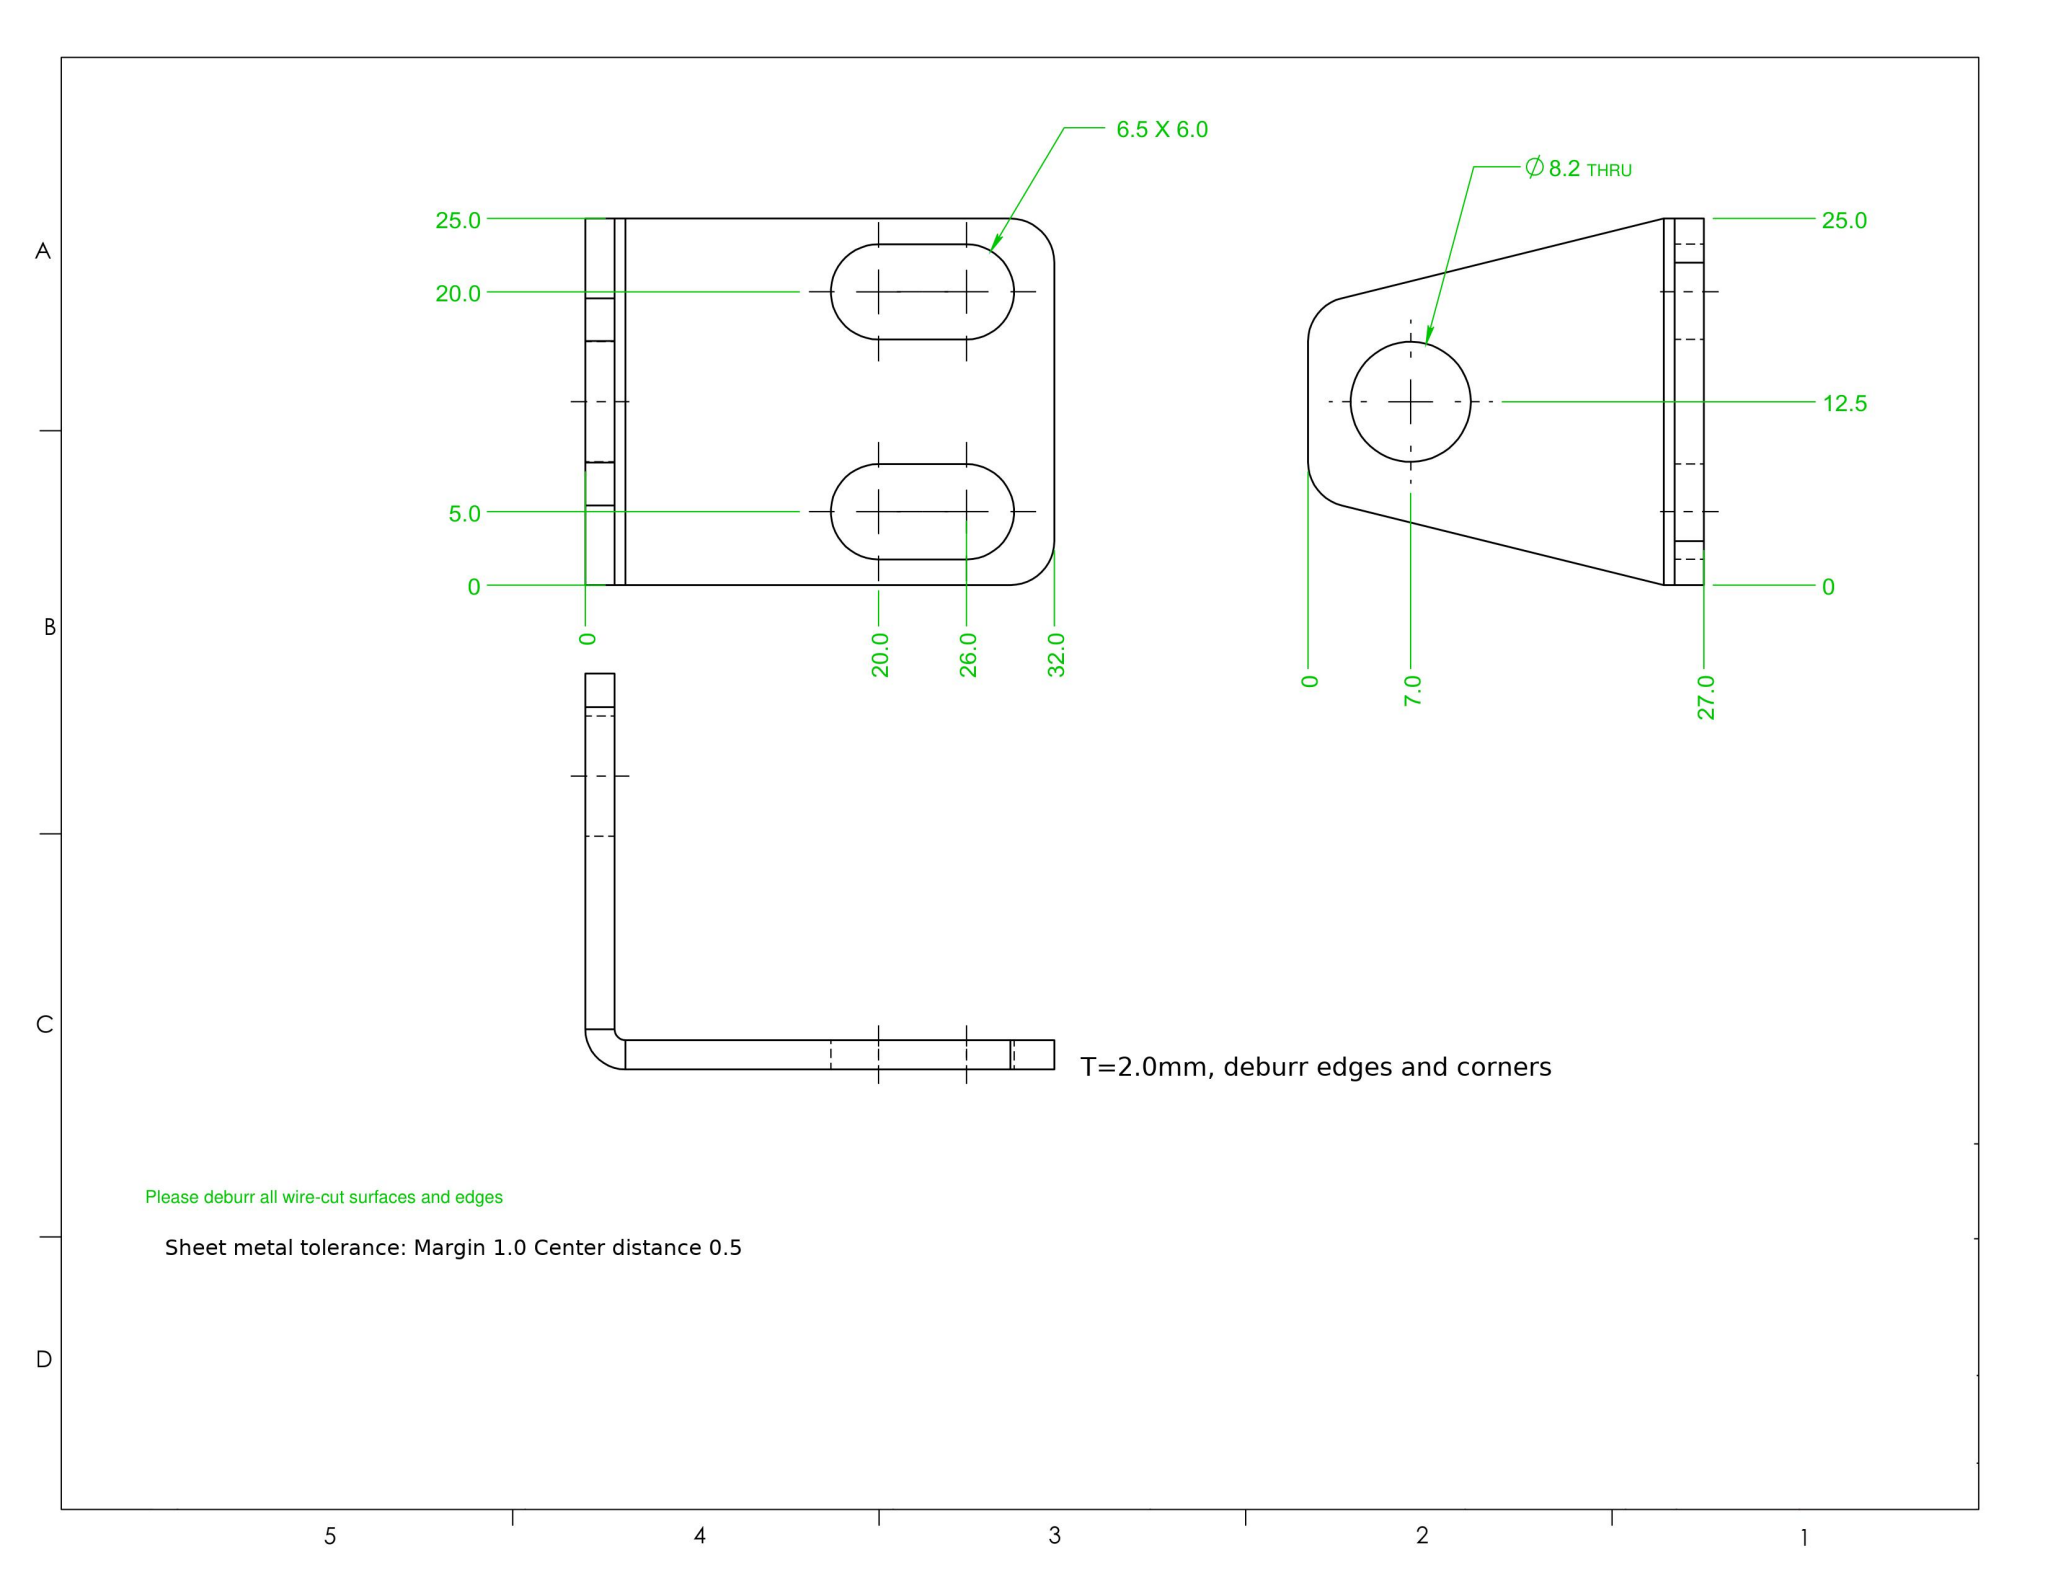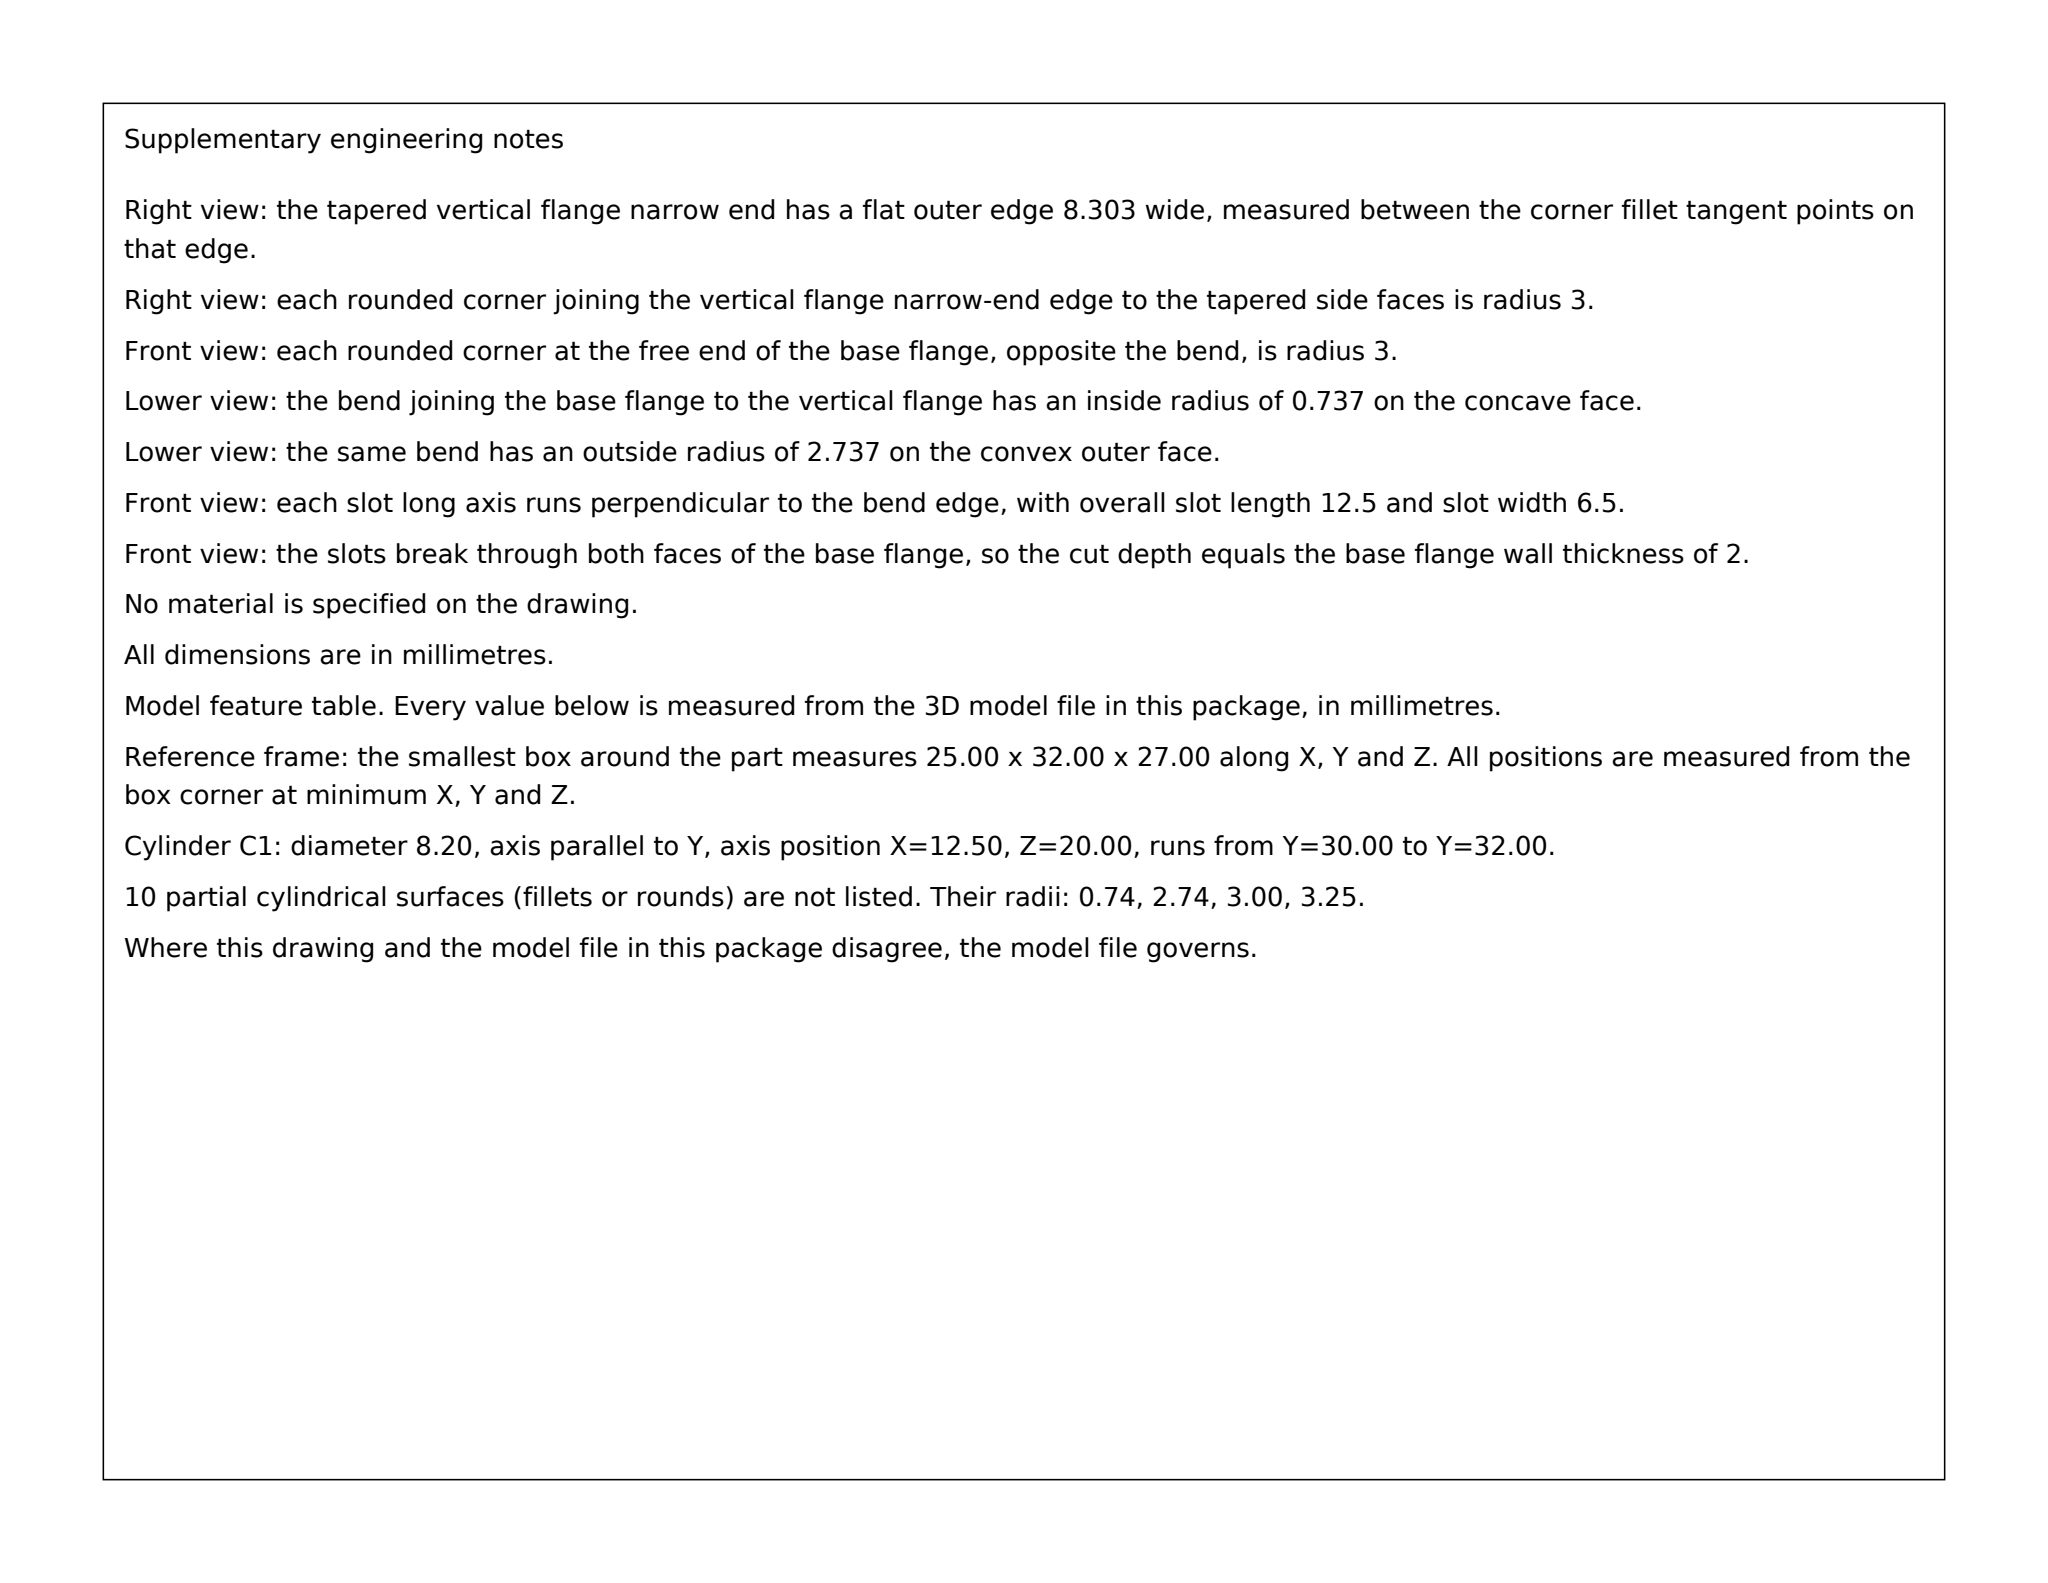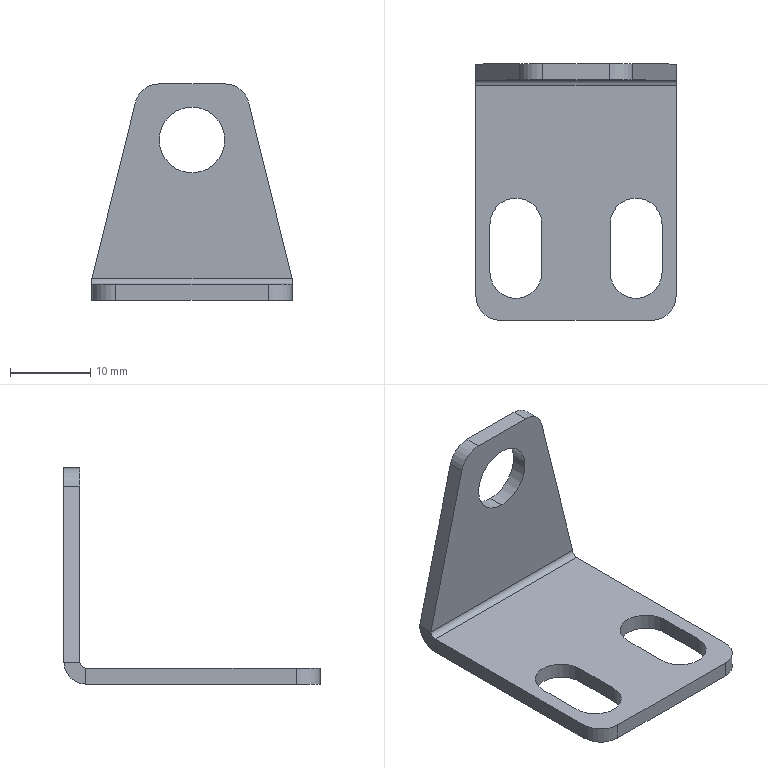Part | SolidWorks | mm | 1 solid | 28 faces | box 25 x 32 x 27 mm | volume 2115 mm3 | plane 16 | cylinder 12 | commonest cylinder face diameters 6 x4 6.5 x4 8.2 x2 5.473 x1 1.473 x1
STEP:
#1=CARTESIAN_POINT('',(12.5,32.,22.1));
#2=VERTEX_POINT('',#1);
#3=CARTESIAN_POINT('',(12.5,32.,13.9));
#4=VERTEX_POINT('',#3);
#5=CARTESIAN_POINT('',(12.5,32.,18.));
#6=DIRECTION('',(0.,-1.,0.));
#7=DIRECTION('',(0.,-0.,-1.));
#8=AXIS2_PLACEMENT_3D('',#5,#6,#7);
#9=CIRCLE('',#8,4.1);
#10=EDGE_CURVE('',#2,#4,#9,.T.);
#11=ORIENTED_EDGE('',*,*,#10,.F.);
#12=CARTESIAN_POINT('',(12.5,30.,22.1));
#13=VERTEX_POINT('',#12);
#14=CARTESIAN_POINT('',(12.5,40.,22.1));
#15=DIRECTION('',(0.,-1.,0.));
#16=VECTOR('',#15,1000.);
#17=LINE('',#14,#16);
#18=EDGE_CURVE('',#2,#13,#17,.T.);
#19=ORIENTED_EDGE('',*,*,#18,.T.);
#20=CARTESIAN_POINT('',(12.5,30.,13.9));
#21=VERTEX_POINT('',#20);
#22=CARTESIAN_POINT('',(12.5,30.,18.));
#23=DIRECTION('',(0.,-1.,0.));
#24=DIRECTION('',(0.,-0.,-1.));
#25=AXIS2_PLACEMENT_3D('',#22,#23,#24);
#26=CIRCLE('',#25,4.1);
#27=EDGE_CURVE('',#13,#21,#26,.T.);
#28=ORIENTED_EDGE('',*,*,#27,.T.);
#29=CARTESIAN_POINT('',(12.5,40.,13.9));
#30=DIRECTION('',(0.,-1.,0.));
#31=VECTOR('',#30,1000.);
#32=LINE('',#29,#31);
#33=EDGE_CURVE('',#4,#21,#32,.T.);
#34=ORIENTED_EDGE('',*,*,#33,.F.);
#35=EDGE_LOOP('',(#11,#19,#28,#34));
#36=FACE_OUTER_BOUND('',#35,.T.);
#37=CARTESIAN_POINT('',(12.5,40.,18.));
#38=DIRECTION('',(0.,-1.,0.));
#39=DIRECTION('',(0.,-0.,-1.));
#40=AXIS2_PLACEMENT_3D('',#37,#38,#39);
#41=CYLINDRICAL_SURFACE('',#40,4.1);
#42=ADVANCED_FACE('',(#36),#41,.F.);
#43=CARTESIAN_POINT('',(12.5,32.,18.));
#44=DIRECTION('',(0.,-1.,0.));
#45=DIRECTION('',(0.,-0.,-1.));
#46=AXIS2_PLACEMENT_3D('',#43,#44,#45);
#47=CIRCLE('',#46,4.1);
#48=EDGE_CURVE('',#4,#2,#47,.T.);
#49=ORIENTED_EDGE('',*,*,#48,.T.);
#50=ORIENTED_EDGE('',*,*,#10,.T.);
#51=EDGE_LOOP('',(#49,#50));
#52=FACE_BOUND('',#51,.T.);
#53=CARTESIAN_POINT('',(0.,32.,0.7366));
#54=VERTEX_POINT('',#53);
#55=CARTESIAN_POINT('',(5.436,32.,22.72));
#56=VERTEX_POINT('',#55);
#57=CARTESIAN_POINT('',(-0.1717,32.,0.04245));
#58=DIRECTION('',(0.2401,0.,0.9708));
#59=VECTOR('',#58,1000.);
#60=LINE('',#57,#59);
#61=EDGE_CURVE('',#54,#56,#60,.T.);
#62=ORIENTED_EDGE('',*,*,#61,.T.);
#63=CARTESIAN_POINT('',(8.349,32.,25.));
#64=VERTEX_POINT('',#63);
#65=CARTESIAN_POINT('',(8.349,32.,22.));
#66=DIRECTION('',(0.,1.,-0.));
#67=DIRECTION('',(0.,-0.,-1.));
#68=AXIS2_PLACEMENT_3D('',#65,#66,#67);
#69=CIRCLE('',#68,3.);
#70=EDGE_CURVE('',#56,#64,#69,.T.);
#71=ORIENTED_EDGE('',*,*,#70,.T.);
#72=CARTESIAN_POINT('',(16.651,32.,25.));
#73=VERTEX_POINT('',#72);
#74=CARTESIAN_POINT('',(25.,32.,25.));
#75=DIRECTION('',(1.,0.,0.));
#76=VECTOR('',#75,1000.);
#77=LINE('',#74,#76);
#78=EDGE_CURVE('',#64,#73,#77,.T.);
#79=ORIENTED_EDGE('',*,*,#78,.T.);
#80=CARTESIAN_POINT('',(19.564,32.,22.72));
#81=VERTEX_POINT('',#80);
#82=CARTESIAN_POINT('',(16.651,32.,22.));
#83=DIRECTION('',(0.,1.,-0.));
#84=DIRECTION('',(-0.,-0.,-1.));
#85=AXIS2_PLACEMENT_3D('',#82,#83,#84);
#86=CIRCLE('',#85,3.);
#87=EDGE_CURVE('',#73,#81,#86,.T.);
#88=ORIENTED_EDGE('',*,*,#87,.T.);
#89=CARTESIAN_POINT('',(25.,32.,0.7366));
#90=VERTEX_POINT('',#89);
#91=CARTESIAN_POINT('',(23.731,32.,5.868));
#92=DIRECTION('',(0.2401,-0.,-0.9708));
#93=VECTOR('',#92,1000.);
#94=LINE('',#91,#93);
#95=EDGE_CURVE('',#81,#90,#94,.T.);
#96=ORIENTED_EDGE('',*,*,#95,.T.);
#97=CARTESIAN_POINT('',(0.,32.,0.7366));
#98=DIRECTION('',(1.,0.,0.));
#99=VECTOR('',#98,1000.);
#100=LINE('',#97,#99);
#101=EDGE_CURVE('',#54,#90,#100,.T.);
#102=ORIENTED_EDGE('',*,*,#101,.F.);
#103=EDGE_LOOP('',(#62,#71,#79,#88,#96,#102));
#104=FACE_OUTER_BOUND('',#103,.T.);
#105=CARTESIAN_POINT('',(0.,32.,-0.));
#106=DIRECTION('',(0.,-1.,0.));
#107=DIRECTION('',(0.,-0.,-1.));
#108=AXIS2_PLACEMENT_3D('',#105,#106,#107);
#109=PLANE('',#108);
#110=ADVANCED_FACE('',(#52,#104),#109,.F.);
#111=CARTESIAN_POINT('',(12.5,30.,18.));
#112=DIRECTION('',(0.,-1.,0.));
#113=DIRECTION('',(0.,-0.,-1.));
#114=AXIS2_PLACEMENT_3D('',#111,#112,#113);
#115=CIRCLE('',#114,4.1);
#116=EDGE_CURVE('',#21,#13,#115,.T.);
#117=ORIENTED_EDGE('',*,*,#116,.F.);
#118=ORIENTED_EDGE('',*,*,#27,.F.);
#119=EDGE_LOOP('',(#117,#118));
#120=FACE_BOUND('',#119,.T.);
#121=CARTESIAN_POINT('',(8.349,30.,25.));
#122=VERTEX_POINT('',#121);
#123=CARTESIAN_POINT('',(16.651,30.,25.));
#124=VERTEX_POINT('',#123);
#125=CARTESIAN_POINT('',(25.,30.,25.));
#126=DIRECTION('',(1.,0.,0.));
#127=VECTOR('',#126,1000.);
#128=LINE('',#125,#127);
#129=EDGE_CURVE('',#122,#124,#128,.T.);
#130=ORIENTED_EDGE('',*,*,#129,.F.);
#131=CARTESIAN_POINT('',(5.436,30.,22.72));
#132=VERTEX_POINT('',#131);
#133=CARTESIAN_POINT('',(8.349,30.,22.));
#134=DIRECTION('',(0.,-1.,0.));
#135=DIRECTION('',(0.,-0.,-1.));
#136=AXIS2_PLACEMENT_3D('',#133,#134,#135);
#137=CIRCLE('',#136,3.);
#138=EDGE_CURVE('',#122,#132,#137,.T.);
#139=ORIENTED_EDGE('',*,*,#138,.T.);
#140=CARTESIAN_POINT('',(-0.,30.,0.7366));
#141=VERTEX_POINT('',#140);
#142=CARTESIAN_POINT('',(-0.1717,30.,0.04245));
#143=DIRECTION('',(0.2401,0.,0.9708));
#144=VECTOR('',#143,1000.);
#145=LINE('',#142,#144);
#146=EDGE_CURVE('',#141,#132,#145,.T.);
#147=ORIENTED_EDGE('',*,*,#146,.F.);
#148=CARTESIAN_POINT('',(25.,30.,0.7366));
#149=VERTEX_POINT('',#148);
#150=CARTESIAN_POINT('',(25.,30.,0.7366));
#151=DIRECTION('',(-1.,0.,0.));
#152=VECTOR('',#151,1000.);
#153=LINE('',#150,#152);
#154=EDGE_CURVE('',#149,#141,#153,.T.);
#155=ORIENTED_EDGE('',*,*,#154,.F.);
#156=CARTESIAN_POINT('',(19.564,30.,22.72));
#157=VERTEX_POINT('',#156);
#158=CARTESIAN_POINT('',(23.731,30.,5.868));
#159=DIRECTION('',(0.2401,-0.,-0.9708));
#160=VECTOR('',#159,1000.);
#161=LINE('',#158,#160);
#162=EDGE_CURVE('',#157,#149,#161,.T.);
#163=ORIENTED_EDGE('',*,*,#162,.F.);
#164=CARTESIAN_POINT('',(16.651,30.,22.));
#165=DIRECTION('',(0.,-1.,0.));
#166=DIRECTION('',(0.,-0.,-1.));
#167=AXIS2_PLACEMENT_3D('',#164,#165,#166);
#168=CIRCLE('',#167,3.);
#169=EDGE_CURVE('',#157,#124,#168,.T.);
#170=ORIENTED_EDGE('',*,*,#169,.T.);
#171=EDGE_LOOP('',(#130,#139,#147,#155,#163,#170));
#172=FACE_OUTER_BOUND('',#171,.T.);
#173=CARTESIAN_POINT('',(0.,30.,-0.));
#174=DIRECTION('',(0.,-1.,0.));
#175=DIRECTION('',(0.,-0.,-1.));
#176=AXIS2_PLACEMENT_3D('',#173,#174,#175);
#177=PLANE('',#176);
#178=ADVANCED_FACE('',(#120,#172),#177,.T.);
#179=ORIENTED_EDGE('',*,*,#78,.F.);
#180=CARTESIAN_POINT('',(8.349,30.,25.));
#181=DIRECTION('',(0.,-1.,0.));
#182=VECTOR('',#181,1000.);
#183=LINE('',#180,#182);
#184=EDGE_CURVE('',#64,#122,#183,.T.);
#185=ORIENTED_EDGE('',*,*,#184,.T.);
#186=ORIENTED_EDGE('',*,*,#129,.T.);
#187=CARTESIAN_POINT('',(16.651,32.,25.));
#188=DIRECTION('',(0.,1.,-0.));
#189=VECTOR('',#188,1000.);
#190=LINE('',#187,#189);
#191=EDGE_CURVE('',#124,#73,#190,.T.);
#192=ORIENTED_EDGE('',*,*,#191,.T.);
#193=EDGE_LOOP('',(#179,#185,#186,#192));
#194=FACE_OUTER_BOUND('',#193,.T.);
#195=CARTESIAN_POINT('',(25.,32.,25.));
#196=DIRECTION('',(0.,-0.,-1.));
#197=DIRECTION('',(0.,1.,-0.));
#198=AXIS2_PLACEMENT_3D('',#195,#196,#197);
#199=PLANE('',#198);
#200=ADVANCED_FACE('',(#194),#199,.F.);
#201=CARTESIAN_POINT('',(0.,29.263,-2.));
#202=VERTEX_POINT('',#201);
#203=CARTESIAN_POINT('',(-0.,3.,-2.));
#204=VERTEX_POINT('',#203);
#205=CARTESIAN_POINT('',(0.,0.,-2.));
#206=DIRECTION('',(0.,-1.,0.));
#207=VECTOR('',#206,1000.);
#208=LINE('',#205,#207);
#209=EDGE_CURVE('',#202,#204,#208,.T.);
#210=ORIENTED_EDGE('',*,*,#209,.T.);
#211=CARTESIAN_POINT('',(-0.,3.,0.));
#212=VERTEX_POINT('',#211);
#213=CARTESIAN_POINT('',(-0.,3.,-2.));
#214=DIRECTION('',(0.,0.,1.));
#215=VECTOR('',#214,1000.);
#216=LINE('',#213,#215);
#217=EDGE_CURVE('',#204,#212,#216,.T.);
#218=ORIENTED_EDGE('',*,*,#217,.T.);
#219=CARTESIAN_POINT('',(0.,29.263,-0.));
#220=VERTEX_POINT('',#219);
#221=CARTESIAN_POINT('',(0.,0.,0.));
#222=DIRECTION('',(0.,-1.,0.));
#223=VECTOR('',#222,1000.);
#224=LINE('',#221,#223);
#225=EDGE_CURVE('',#220,#212,#224,.T.);
#226=ORIENTED_EDGE('',*,*,#225,.F.);
#227=CARTESIAN_POINT('',(0.,29.263,-0.));
#228=DIRECTION('',(0.,0.,-1.));
#229=VECTOR('',#228,1000.);
#230=LINE('',#227,#229);
#231=EDGE_CURVE('',#220,#202,#230,.T.);
#232=ORIENTED_EDGE('',*,*,#231,.T.);
#233=EDGE_LOOP('',(#210,#218,#226,#232));
#234=FACE_OUTER_BOUND('',#233,.T.);
#235=CARTESIAN_POINT('',(0.,0.,-2.));
#236=DIRECTION('',(-1.,-0.,0.));
#237=DIRECTION('',(0.,-1.,0.));
#238=AXIS2_PLACEMENT_3D('',#235,#236,#237);
#239=PLANE('',#238);
#240=ADVANCED_FACE('',(#234),#239,.T.);
#241=CARTESIAN_POINT('',(23.25,12.,-2.));
#242=VERTEX_POINT('',#241);
#243=CARTESIAN_POINT('',(16.75,12.,-2.));
#244=VERTEX_POINT('',#243);
#245=CARTESIAN_POINT('',(20.,12.,-2.));
#246=DIRECTION('',(0.,0.,1.));
#247=DIRECTION('',(1.,0.,0.));
#248=AXIS2_PLACEMENT_3D('',#245,#246,#247);
#249=CIRCLE('',#248,3.25);
#250=EDGE_CURVE('',#242,#244,#249,.T.);
#251=ORIENTED_EDGE('',*,*,#250,.T.);
#252=CARTESIAN_POINT('',(16.75,6.,-2.));
#253=VERTEX_POINT('',#252);
#254=CARTESIAN_POINT('',(16.75,12.,-2.));
#255=DIRECTION('',(0.,-1.,0.));
#256=VECTOR('',#255,1000.);
#257=LINE('',#254,#256);
#258=EDGE_CURVE('',#244,#253,#257,.T.);
#259=ORIENTED_EDGE('',*,*,#258,.T.);
#260=CARTESIAN_POINT('',(23.25,6.,-2.));
#261=VERTEX_POINT('',#260);
#262=CARTESIAN_POINT('',(20.,6.,-2.));
#263=DIRECTION('',(0.,0.,1.));
#264=DIRECTION('',(1.,0.,0.));
#265=AXIS2_PLACEMENT_3D('',#262,#263,#264);
#266=CIRCLE('',#265,3.25);
#267=EDGE_CURVE('',#253,#261,#266,.T.);
#268=ORIENTED_EDGE('',*,*,#267,.T.);
#269=CARTESIAN_POINT('',(23.25,12.,-2.));
#270=DIRECTION('',(-0.,1.,0.));
#271=VECTOR('',#270,1000.);
#272=LINE('',#269,#271);
#273=EDGE_CURVE('',#261,#242,#272,.T.);
#274=ORIENTED_EDGE('',*,*,#273,.T.);
#275=EDGE_LOOP('',(#251,#259,#268,#274));
#276=FACE_BOUND('',#275,.T.);
#277=CARTESIAN_POINT('',(8.25,12.,-2.));
#278=VERTEX_POINT('',#277);
#279=CARTESIAN_POINT('',(1.75,12.,-2.));
#280=VERTEX_POINT('',#279);
#281=CARTESIAN_POINT('',(5.,12.,-2.));
#282=DIRECTION('',(0.,0.,1.));
#283=DIRECTION('',(1.,0.,0.));
#284=AXIS2_PLACEMENT_3D('',#281,#282,#283);
#285=CIRCLE('',#284,3.25);
#286=EDGE_CURVE('',#278,#280,#285,.T.);
#287=ORIENTED_EDGE('',*,*,#286,.T.);
#288=CARTESIAN_POINT('',(1.75,6.,-2.));
#289=VERTEX_POINT('',#288);
#290=CARTESIAN_POINT('',(1.75,12.,-2.));
#291=DIRECTION('',(0.,-1.,0.));
#292=VECTOR('',#291,1000.);
#293=LINE('',#290,#292);
#294=EDGE_CURVE('',#280,#289,#293,.T.);
#295=ORIENTED_EDGE('',*,*,#294,.T.);
#296=CARTESIAN_POINT('',(8.25,6.,-2.));
#297=VERTEX_POINT('',#296);
#298=CARTESIAN_POINT('',(5.,6.,-2.));
#299=DIRECTION('',(0.,0.,1.));
#300=DIRECTION('',(1.,0.,0.));
#301=AXIS2_PLACEMENT_3D('',#298,#299,#300);
#302=CIRCLE('',#301,3.25);
#303=EDGE_CURVE('',#289,#297,#302,.T.);
#304=ORIENTED_EDGE('',*,*,#303,.T.);
#305=CARTESIAN_POINT('',(8.25,12.,-2.));
#306=DIRECTION('',(-0.,1.,0.));
#307=VECTOR('',#306,1000.);
#308=LINE('',#305,#307);
#309=EDGE_CURVE('',#297,#278,#308,.T.);
#310=ORIENTED_EDGE('',*,*,#309,.T.);
#311=EDGE_LOOP('',(#287,#295,#304,#310));
#312=FACE_BOUND('',#311,.T.);
#313=CARTESIAN_POINT('',(3.,0.,-2.));
#314=VERTEX_POINT('',#313);
#315=CARTESIAN_POINT('',(22.,0.,-2.));
#316=VERTEX_POINT('',#315);
#317=CARTESIAN_POINT('',(0.,0.,-2.));
#318=DIRECTION('',(1.,0.,0.));
#319=VECTOR('',#318,1000.);
#320=LINE('',#317,#319);
#321=EDGE_CURVE('',#314,#316,#320,.T.);
#322=ORIENTED_EDGE('',*,*,#321,.F.);
#323=CARTESIAN_POINT('',(3.,3.,-2.));
#324=DIRECTION('',(0.,0.,-1.));
#325=DIRECTION('',(-1.,0.,0.));
#326=AXIS2_PLACEMENT_3D('',#323,#324,#325);
#327=CIRCLE('',#326,3.);
#328=EDGE_CURVE('',#314,#204,#327,.T.);
#329=ORIENTED_EDGE('',*,*,#328,.T.);
#330=ORIENTED_EDGE('',*,*,#209,.F.);
#331=CARTESIAN_POINT('',(25.,29.263,-2.));
#332=VERTEX_POINT('',#331);
#333=CARTESIAN_POINT('',(-0.,29.263,-2.));
#334=DIRECTION('',(1.,0.,0.));
#335=VECTOR('',#334,1000.);
#336=LINE('',#333,#335);
#337=EDGE_CURVE('',#202,#332,#336,.T.);
#338=ORIENTED_EDGE('',*,*,#337,.T.);
#339=CARTESIAN_POINT('',(25.,3.,-2.));
#340=VERTEX_POINT('',#339);
#341=CARTESIAN_POINT('',(25.,0.,-2.));
#342=DIRECTION('',(-0.,1.,0.));
#343=VECTOR('',#342,1000.);
#344=LINE('',#341,#343);
#345=EDGE_CURVE('',#340,#332,#344,.T.);
#346=ORIENTED_EDGE('',*,*,#345,.F.);
#347=CARTESIAN_POINT('',(22.,3.,-2.));
#348=DIRECTION('',(0.,0.,-1.));
#349=DIRECTION('',(-1.,0.,0.));
#350=AXIS2_PLACEMENT_3D('',#347,#348,#349);
#351=CIRCLE('',#350,3.);
#352=EDGE_CURVE('',#340,#316,#351,.T.);
#353=ORIENTED_EDGE('',*,*,#352,.T.);
#354=EDGE_LOOP('',(#322,#329,#330,#338,#346,#353));
#355=FACE_OUTER_BOUND('',#354,.T.);
#356=CARTESIAN_POINT('',(0.,0.,-2.));
#357=DIRECTION('',(0.,0.,-1.));
#358=DIRECTION('',(-1.,0.,0.));
#359=AXIS2_PLACEMENT_3D('',#356,#357,#358);
#360=PLANE('',#359);
#361=ADVANCED_FACE('',(#276,#312,#355),#360,.T.);
#362=CARTESIAN_POINT('',(16.75,12.,0.));
#363=VERTEX_POINT('',#362);
#364=CARTESIAN_POINT('',(16.75,6.,0.));
#365=VERTEX_POINT('',#364);
#366=CARTESIAN_POINT('',(16.75,12.,0.));
#367=DIRECTION('',(0.,-1.,0.));
#368=VECTOR('',#367,1000.);
#369=LINE('',#366,#368);
#370=EDGE_CURVE('',#363,#365,#369,.T.);
#371=ORIENTED_EDGE('',*,*,#370,.F.);
#372=CARTESIAN_POINT('',(23.25,12.,0.));
#373=VERTEX_POINT('',#372);
#374=CARTESIAN_POINT('',(20.,12.,0.));
#375=DIRECTION('',(0.,0.,1.));
#376=DIRECTION('',(1.,0.,0.));
#377=AXIS2_PLACEMENT_3D('',#374,#375,#376);
#378=CIRCLE('',#377,3.25);
#379=EDGE_CURVE('',#373,#363,#378,.T.);
#380=ORIENTED_EDGE('',*,*,#379,.F.);
#381=CARTESIAN_POINT('',(23.25,6.,0.));
#382=VERTEX_POINT('',#381);
#383=CARTESIAN_POINT('',(23.25,12.,0.));
#384=DIRECTION('',(-0.,1.,0.));
#385=VECTOR('',#384,1000.);
#386=LINE('',#383,#385);
#387=EDGE_CURVE('',#382,#373,#386,.T.);
#388=ORIENTED_EDGE('',*,*,#387,.F.);
#389=CARTESIAN_POINT('',(20.,6.,0.));
#390=DIRECTION('',(0.,0.,1.));
#391=DIRECTION('',(1.,0.,0.));
#392=AXIS2_PLACEMENT_3D('',#389,#390,#391);
#393=CIRCLE('',#392,3.25);
#394=EDGE_CURVE('',#365,#382,#393,.T.);
#395=ORIENTED_EDGE('',*,*,#394,.F.);
#396=EDGE_LOOP('',(#371,#380,#388,#395));
#397=FACE_BOUND('',#396,.T.);
#398=CARTESIAN_POINT('',(1.75,12.,0.));
#399=VERTEX_POINT('',#398);
#400=CARTESIAN_POINT('',(1.75,6.,0.));
#401=VERTEX_POINT('',#400);
#402=CARTESIAN_POINT('',(1.75,12.,0.));
#403=DIRECTION('',(0.,-1.,0.));
#404=VECTOR('',#403,1000.);
#405=LINE('',#402,#404);
#406=EDGE_CURVE('',#399,#401,#405,.T.);
#407=ORIENTED_EDGE('',*,*,#406,.F.);
#408=CARTESIAN_POINT('',(8.25,12.,0.));
#409=VERTEX_POINT('',#408);
#410=CARTESIAN_POINT('',(5.,12.,0.));
#411=DIRECTION('',(0.,0.,1.));
#412=DIRECTION('',(1.,0.,0.));
#413=AXIS2_PLACEMENT_3D('',#410,#411,#412);
#414=CIRCLE('',#413,3.25);
#415=EDGE_CURVE('',#409,#399,#414,.T.);
#416=ORIENTED_EDGE('',*,*,#415,.F.);
#417=CARTESIAN_POINT('',(8.25,6.,0.));
#418=VERTEX_POINT('',#417);
#419=CARTESIAN_POINT('',(8.25,12.,0.));
#420=DIRECTION('',(-0.,1.,0.));
#421=VECTOR('',#420,1000.);
#422=LINE('',#419,#421);
#423=EDGE_CURVE('',#418,#409,#422,.T.);
#424=ORIENTED_EDGE('',*,*,#423,.F.);
#425=CARTESIAN_POINT('',(5.,6.,0.));
#426=DIRECTION('',(0.,0.,1.));
#427=DIRECTION('',(1.,0.,0.));
#428=AXIS2_PLACEMENT_3D('',#425,#426,#427);
#429=CIRCLE('',#428,3.25);
#430=EDGE_CURVE('',#401,#418,#429,.T.);
#431=ORIENTED_EDGE('',*,*,#430,.F.);
#432=EDGE_LOOP('',(#407,#416,#424,#431));
#433=FACE_BOUND('',#432,.T.);
#434=ORIENTED_EDGE('',*,*,#225,.T.);
#435=CARTESIAN_POINT('',(3.,0.,0.));
#436=VERTEX_POINT('',#435);
#437=CARTESIAN_POINT('',(3.,3.,0.));
#438=DIRECTION('',(0.,0.,1.));
#439=DIRECTION('',(-1.,0.,0.));
#440=AXIS2_PLACEMENT_3D('',#437,#438,#439);
#441=CIRCLE('',#440,3.);
#442=EDGE_CURVE('',#212,#436,#441,.T.);
#443=ORIENTED_EDGE('',*,*,#442,.T.);
#444=CARTESIAN_POINT('',(22.,0.,0.));
#445=VERTEX_POINT('',#444);
#446=CARTESIAN_POINT('',(0.,0.,0.));
#447=DIRECTION('',(1.,0.,0.));
#448=VECTOR('',#447,1000.);
#449=LINE('',#446,#448);
#450=EDGE_CURVE('',#436,#445,#449,.T.);
#451=ORIENTED_EDGE('',*,*,#450,.T.);
#452=CARTESIAN_POINT('',(25.,3.,0.));
#453=VERTEX_POINT('',#452);
#454=CARTESIAN_POINT('',(22.,3.,0.));
#455=DIRECTION('',(0.,0.,1.));
#456=DIRECTION('',(-1.,0.,0.));
#457=AXIS2_PLACEMENT_3D('',#454,#455,#456);
#458=CIRCLE('',#457,3.);
#459=EDGE_CURVE('',#445,#453,#458,.T.);
#460=ORIENTED_EDGE('',*,*,#459,.T.);
#461=CARTESIAN_POINT('',(25.,29.263,-0.));
#462=VERTEX_POINT('',#461);
#463=CARTESIAN_POINT('',(25.,0.,0.));
#464=DIRECTION('',(-0.,1.,0.));
#465=VECTOR('',#464,1000.);
#466=LINE('',#463,#465);
#467=EDGE_CURVE('',#453,#462,#466,.T.);
#468=ORIENTED_EDGE('',*,*,#467,.T.);
#469=CARTESIAN_POINT('',(-0.,29.263,-0.));
#470=DIRECTION('',(1.,0.,0.));
#471=VECTOR('',#470,1000.);
#472=LINE('',#469,#471);
#473=EDGE_CURVE('',#220,#462,#472,.T.);
#474=ORIENTED_EDGE('',*,*,#473,.F.);
#475=EDGE_LOOP('',(#434,#443,#451,#460,#468,#474));
#476=FACE_OUTER_BOUND('',#475,.T.);
#477=CARTESIAN_POINT('',(0.,0.,0.));
#478=DIRECTION('',(0.,0.,-1.));
#479=DIRECTION('',(-1.,0.,0.));
#480=AXIS2_PLACEMENT_3D('',#477,#478,#479);
#481=PLANE('',#480);
#482=ADVANCED_FACE('',(#397,#433,#476),#481,.F.);
#483=ORIENTED_EDGE('',*,*,#467,.F.);
#484=CARTESIAN_POINT('',(25.,3.,-2.));
#485=DIRECTION('',(0.,0.,-1.));
#486=VECTOR('',#485,1000.);
#487=LINE('',#484,#486);
#488=EDGE_CURVE('',#453,#340,#487,.T.);
#489=ORIENTED_EDGE('',*,*,#488,.T.);
#490=ORIENTED_EDGE('',*,*,#345,.T.);
#491=CARTESIAN_POINT('',(25.,29.263,-0.));
#492=DIRECTION('',(0.,0.,-1.));
#493=VECTOR('',#492,1000.);
#494=LINE('',#491,#493);
#495=EDGE_CURVE('',#462,#332,#494,.T.);
#496=ORIENTED_EDGE('',*,*,#495,.F.);
#497=EDGE_LOOP('',(#483,#489,#490,#496));
#498=FACE_OUTER_BOUND('',#497,.T.);
#499=CARTESIAN_POINT('',(25.,0.,-2.));
#500=DIRECTION('',(1.,0.,0.));
#501=DIRECTION('',(-0.,1.,0.));
#502=AXIS2_PLACEMENT_3D('',#499,#500,#501);
#503=PLANE('',#502);
#504=ADVANCED_FACE('',(#498),#503,.T.);
#505=ORIENTED_EDGE('',*,*,#450,.F.);
#506=CARTESIAN_POINT('',(3.,0.,-2.));
#507=DIRECTION('',(0.,0.,-1.));
#508=VECTOR('',#507,1000.);
#509=LINE('',#506,#508);
#510=EDGE_CURVE('',#436,#314,#509,.T.);
#511=ORIENTED_EDGE('',*,*,#510,.T.);
#512=ORIENTED_EDGE('',*,*,#321,.T.);
#513=CARTESIAN_POINT('',(22.,0.,-2.));
#514=DIRECTION('',(0.,0.,1.));
#515=VECTOR('',#514,1000.);
#516=LINE('',#513,#515);
#517=EDGE_CURVE('',#316,#445,#516,.T.);
#518=ORIENTED_EDGE('',*,*,#517,.T.);
#519=EDGE_LOOP('',(#505,#511,#512,#518));
#520=FACE_OUTER_BOUND('',#519,.T.);
#521=CARTESIAN_POINT('',(0.,0.,-2.));
#522=DIRECTION('',(0.,-1.,0.));
#523=DIRECTION('',(0.,0.,-1.));
#524=AXIS2_PLACEMENT_3D('',#521,#522,#523);
#525=PLANE('',#524);
#526=ADVANCED_FACE('',(#520),#525,.T.);
#527=CARTESIAN_POINT('',(25.,30.,0.7366));
#528=DIRECTION('',(0.,1.,-0.));
#529=VECTOR('',#528,1000.);
#530=LINE('',#527,#529);
#531=EDGE_CURVE('',#149,#90,#530,.T.);
#532=ORIENTED_EDGE('',*,*,#531,.F.);
#533=CARTESIAN_POINT('',(25.,29.263,0.7366));
#534=DIRECTION('',(1.,0.,0.));
#535=DIRECTION('',(0.,0.,1.));
#536=AXIS2_PLACEMENT_3D('',#533,#534,#535);
#537=CIRCLE('',#536,0.7366);
#538=EDGE_CURVE('',#462,#149,#537,.T.);
#539=ORIENTED_EDGE('',*,*,#538,.F.);
#540=ORIENTED_EDGE('',*,*,#495,.T.);
#541=CARTESIAN_POINT('',(25.,29.263,0.7366));
#542=DIRECTION('',(1.,0.,0.));
#543=DIRECTION('',(0.,0.,1.));
#544=AXIS2_PLACEMENT_3D('',#541,#542,#543);
#545=CIRCLE('',#544,2.737);
#546=EDGE_CURVE('',#332,#90,#545,.T.);
#547=ORIENTED_EDGE('',*,*,#546,.T.);
#548=EDGE_LOOP('',(#532,#539,#540,#547));
#549=FACE_OUTER_BOUND('',#548,.T.);
#550=CARTESIAN_POINT('',(25.,29.263,0.7366));
#551=DIRECTION('',(1.,0.,0.));
#552=DIRECTION('',(0.,0.,-1.));
#553=AXIS2_PLACEMENT_3D('',#550,#551,#552);
#554=PLANE('',#553);
#555=ADVANCED_FACE('',(#549),#554,.T.);
#556=CARTESIAN_POINT('',(0.,29.263,0.7366));
#557=DIRECTION('',(-1.,0.,0.));
#558=DIRECTION('',(0.,0.,1.));
#559=AXIS2_PLACEMENT_3D('',#556,#557,#558);
#560=CIRCLE('',#559,0.7366);
#561=EDGE_CURVE('',#141,#220,#560,.T.);
#562=ORIENTED_EDGE('',*,*,#561,.F.);
#563=CARTESIAN_POINT('',(0.,30.,0.7366));
#564=DIRECTION('',(0.,1.,-0.));
#565=VECTOR('',#564,1000.);
#566=LINE('',#563,#565);
#567=EDGE_CURVE('',#141,#54,#566,.T.);
#568=ORIENTED_EDGE('',*,*,#567,.T.);
#569=CARTESIAN_POINT('',(0.,29.263,0.7366));
#570=DIRECTION('',(-1.,0.,0.));
#571=DIRECTION('',(0.,0.,1.));
#572=AXIS2_PLACEMENT_3D('',#569,#570,#571);
#573=CIRCLE('',#572,2.737);
#574=EDGE_CURVE('',#54,#202,#573,.T.);
#575=ORIENTED_EDGE('',*,*,#574,.T.);
#576=ORIENTED_EDGE('',*,*,#231,.F.);
#577=EDGE_LOOP('',(#562,#568,#575,#576));
#578=FACE_OUTER_BOUND('',#577,.T.);
#579=CARTESIAN_POINT('',(0.,29.263,0.7366));
#580=DIRECTION('',(1.,0.,0.));
#581=DIRECTION('',(0.,0.,-1.));
#582=AXIS2_PLACEMENT_3D('',#579,#580,#581);
#583=PLANE('',#582);
#584=ADVANCED_FACE('',(#578),#583,.F.);
#585=ORIENTED_EDGE('',*,*,#337,.F.);
#586=ORIENTED_EDGE('',*,*,#574,.F.);
#587=ORIENTED_EDGE('',*,*,#101,.T.);
#588=ORIENTED_EDGE('',*,*,#546,.F.);
#589=EDGE_LOOP('',(#585,#586,#587,#588));
#590=FACE_OUTER_BOUND('',#589,.T.);
#591=CARTESIAN_POINT('',(-0.,29.263,0.7366));
#592=DIRECTION('',(-1.,0.,0.));
#593=DIRECTION('',(0.,1.,-0.));
#594=AXIS2_PLACEMENT_3D('',#591,#592,#593);
#595=CYLINDRICAL_SURFACE('',#594,2.737);
#596=ADVANCED_FACE('',(#590),#595,.T.);
#597=ORIENTED_EDGE('',*,*,#473,.T.);
#598=ORIENTED_EDGE('',*,*,#538,.T.);
#599=ORIENTED_EDGE('',*,*,#154,.T.);
#600=ORIENTED_EDGE('',*,*,#561,.T.);
#601=EDGE_LOOP('',(#597,#598,#599,#600));
#602=FACE_OUTER_BOUND('',#601,.T.);
#603=CARTESIAN_POINT('',(-0.,29.263,0.7366));
#604=DIRECTION('',(-1.,0.,0.));
#605=DIRECTION('',(0.,1.,-0.));
#606=AXIS2_PLACEMENT_3D('',#603,#604,#605);
#607=CYLINDRICAL_SURFACE('',#606,0.7366);
#608=ADVANCED_FACE('',(#602),#607,.F.);
#609=ORIENTED_EDGE('',*,*,#95,.F.);
#610=CARTESIAN_POINT('',(19.564,30.,22.72));
#611=DIRECTION('',(-0.,-1.,0.));
#612=VECTOR('',#611,1000.);
#613=LINE('',#610,#612);
#614=EDGE_CURVE('',#81,#157,#613,.T.);
#615=ORIENTED_EDGE('',*,*,#614,.T.);
#616=ORIENTED_EDGE('',*,*,#162,.T.);
#617=ORIENTED_EDGE('',*,*,#531,.T.);
#618=EDGE_LOOP('',(#609,#615,#616,#617));
#619=FACE_OUTER_BOUND('',#618,.T.);
#620=CARTESIAN_POINT('',(23.731,32.,5.868));
#621=DIRECTION('',(-0.9708,-0.,-0.2401));
#622=DIRECTION('',(0.2401,-0.,-0.9708));
#623=AXIS2_PLACEMENT_3D('',#620,#621,#622);
#624=PLANE('',#623);
#625=ADVANCED_FACE('',(#619),#624,.F.);
#626=ORIENTED_EDGE('',*,*,#146,.T.);
#627=CARTESIAN_POINT('',(5.436,32.,22.72));
#628=DIRECTION('',(-0.,1.,-0.));
#629=VECTOR('',#628,1000.);
#630=LINE('',#627,#629);
#631=EDGE_CURVE('',#132,#56,#630,.T.);
#632=ORIENTED_EDGE('',*,*,#631,.T.);
#633=ORIENTED_EDGE('',*,*,#61,.F.);
#634=ORIENTED_EDGE('',*,*,#567,.F.);
#635=EDGE_LOOP('',(#626,#632,#633,#634));
#636=FACE_OUTER_BOUND('',#635,.T.);
#637=CARTESIAN_POINT('',(-0.1717,32.,0.04245));
#638=DIRECTION('',(0.9708,-0.,-0.2401));
#639=DIRECTION('',(0.2401,0.,0.9708));
#640=AXIS2_PLACEMENT_3D('',#637,#638,#639);
#641=PLANE('',#640);
#642=ADVANCED_FACE('',(#636),#641,.F.);
#643=ORIENTED_EDGE('',*,*,#328,.F.);
#644=ORIENTED_EDGE('',*,*,#510,.F.);
#645=ORIENTED_EDGE('',*,*,#442,.F.);
#646=ORIENTED_EDGE('',*,*,#217,.F.);
#647=EDGE_LOOP('',(#643,#644,#645,#646));
#648=FACE_OUTER_BOUND('',#647,.T.);
#649=CARTESIAN_POINT('',(3.,3.,-2.));
#650=DIRECTION('',(0.,0.,1.));
#651=DIRECTION('',(1.,0.,0.));
#652=AXIS2_PLACEMENT_3D('',#649,#650,#651);
#653=CYLINDRICAL_SURFACE('',#652,3.);
#654=ADVANCED_FACE('',(#648),#653,.T.);
#655=ORIENTED_EDGE('',*,*,#352,.F.);
#656=ORIENTED_EDGE('',*,*,#488,.F.);
#657=ORIENTED_EDGE('',*,*,#459,.F.);
#658=ORIENTED_EDGE('',*,*,#517,.F.);
#659=EDGE_LOOP('',(#655,#656,#657,#658));
#660=FACE_OUTER_BOUND('',#659,.T.);
#661=CARTESIAN_POINT('',(22.,3.,-2.));
#662=DIRECTION('',(0.,0.,1.));
#663=DIRECTION('',(1.,0.,0.));
#664=AXIS2_PLACEMENT_3D('',#661,#662,#663);
#665=CYLINDRICAL_SURFACE('',#664,3.);
#666=ADVANCED_FACE('',(#660),#665,.T.);
#667=ORIENTED_EDGE('',*,*,#70,.F.);
#668=ORIENTED_EDGE('',*,*,#631,.F.);
#669=ORIENTED_EDGE('',*,*,#138,.F.);
#670=ORIENTED_EDGE('',*,*,#184,.F.);
#671=EDGE_LOOP('',(#667,#668,#669,#670));
#672=FACE_OUTER_BOUND('',#671,.T.);
#673=CARTESIAN_POINT('',(8.349,32.,22.));
#674=DIRECTION('',(0.,-1.,0.));
#675=DIRECTION('',(0.,-0.,-1.));
#676=AXIS2_PLACEMENT_3D('',#673,#674,#675);
#677=CYLINDRICAL_SURFACE('',#676,3.);
#678=ADVANCED_FACE('',(#672),#677,.T.);
#679=ORIENTED_EDGE('',*,*,#87,.F.);
#680=ORIENTED_EDGE('',*,*,#191,.F.);
#681=ORIENTED_EDGE('',*,*,#169,.F.);
#682=ORIENTED_EDGE('',*,*,#614,.F.);
#683=EDGE_LOOP('',(#679,#680,#681,#682));
#684=FACE_OUTER_BOUND('',#683,.T.);
#685=CARTESIAN_POINT('',(16.651,32.,22.));
#686=DIRECTION('',(-0.,-1.,0.));
#687=DIRECTION('',(0.,-0.,-1.));
#688=AXIS2_PLACEMENT_3D('',#685,#686,#687);
#689=CYLINDRICAL_SURFACE('',#688,3.);
#690=ADVANCED_FACE('',(#684),#689,.T.);
#691=ORIENTED_EDGE('',*,*,#18,.F.);
#692=ORIENTED_EDGE('',*,*,#48,.F.);
#693=ORIENTED_EDGE('',*,*,#33,.T.);
#694=ORIENTED_EDGE('',*,*,#116,.T.);
#695=EDGE_LOOP('',(#691,#692,#693,#694));
#696=FACE_OUTER_BOUND('',#695,.T.);
#697=CARTESIAN_POINT('',(12.5,40.,18.));
#698=DIRECTION('',(0.,-1.,0.));
#699=DIRECTION('',(0.,-0.,-1.));
#700=AXIS2_PLACEMENT_3D('',#697,#698,#699);
#701=CYLINDRICAL_SURFACE('',#700,4.1);
#702=ADVANCED_FACE('',(#696),#701,.F.);
#703=ORIENTED_EDGE('',*,*,#415,.T.);
#704=CARTESIAN_POINT('',(1.75,12.,-2.));
#705=DIRECTION('',(0.,0.,1.));
#706=VECTOR('',#705,1000.);
#707=LINE('',#704,#706);
#708=EDGE_CURVE('',#280,#399,#707,.T.);
#709=ORIENTED_EDGE('',*,*,#708,.F.);
#710=ORIENTED_EDGE('',*,*,#286,.F.);
#711=CARTESIAN_POINT('',(8.25,12.,-2.));
#712=DIRECTION('',(0.,0.,1.));
#713=VECTOR('',#712,1000.);
#714=LINE('',#711,#713);
#715=EDGE_CURVE('',#278,#409,#714,.T.);
#716=ORIENTED_EDGE('',*,*,#715,.T.);
#717=EDGE_LOOP('',(#703,#709,#710,#716));
#718=FACE_OUTER_BOUND('',#717,.T.);
#719=CARTESIAN_POINT('',(5.,12.,-2.));
#720=DIRECTION('',(0.,0.,1.));
#721=DIRECTION('',(1.,0.,0.));
#722=AXIS2_PLACEMENT_3D('',#719,#720,#721);
#723=CYLINDRICAL_SURFACE('',#722,3.25);
#724=ADVANCED_FACE('',(#718),#723,.F.);
#725=ORIENTED_EDGE('',*,*,#423,.T.);
#726=ORIENTED_EDGE('',*,*,#715,.F.);
#727=ORIENTED_EDGE('',*,*,#309,.F.);
#728=CARTESIAN_POINT('',(8.25,6.,-2.));
#729=DIRECTION('',(0.,0.,1.));
#730=VECTOR('',#729,1000.);
#731=LINE('',#728,#730);
#732=EDGE_CURVE('',#297,#418,#731,.T.);
#733=ORIENTED_EDGE('',*,*,#732,.T.);
#734=EDGE_LOOP('',(#725,#726,#727,#733));
#735=FACE_OUTER_BOUND('',#734,.T.);
#736=CARTESIAN_POINT('',(8.25,12.,-2.));
#737=DIRECTION('',(1.,0.,0.));
#738=DIRECTION('',(-0.,1.,0.));
#739=AXIS2_PLACEMENT_3D('',#736,#737,#738);
#740=PLANE('',#739);
#741=ADVANCED_FACE('',(#735),#740,.F.);
#742=ORIENTED_EDGE('',*,*,#430,.T.);
#743=ORIENTED_EDGE('',*,*,#732,.F.);
#744=ORIENTED_EDGE('',*,*,#303,.F.);
#745=CARTESIAN_POINT('',(1.75,6.,-2.));
#746=DIRECTION('',(0.,0.,1.));
#747=VECTOR('',#746,1000.);
#748=LINE('',#745,#747);
#749=EDGE_CURVE('',#289,#401,#748,.T.);
#750=ORIENTED_EDGE('',*,*,#749,.T.);
#751=EDGE_LOOP('',(#742,#743,#744,#750));
#752=FACE_OUTER_BOUND('',#751,.T.);
#753=CARTESIAN_POINT('',(5.,6.,-2.));
#754=DIRECTION('',(0.,0.,1.));
#755=DIRECTION('',(1.,0.,0.));
#756=AXIS2_PLACEMENT_3D('',#753,#754,#755);
#757=CYLINDRICAL_SURFACE('',#756,3.25);
#758=ADVANCED_FACE('',(#752),#757,.F.);
#759=ORIENTED_EDGE('',*,*,#406,.T.);
#760=ORIENTED_EDGE('',*,*,#749,.F.);
#761=ORIENTED_EDGE('',*,*,#294,.F.);
#762=ORIENTED_EDGE('',*,*,#708,.T.);
#763=EDGE_LOOP('',(#759,#760,#761,#762));
#764=FACE_OUTER_BOUND('',#763,.T.);
#765=CARTESIAN_POINT('',(1.75,12.,-2.));
#766=DIRECTION('',(-1.,-0.,0.));
#767=DIRECTION('',(0.,-1.,0.));
#768=AXIS2_PLACEMENT_3D('',#765,#766,#767);
#769=PLANE('',#768);
#770=ADVANCED_FACE('',(#764),#769,.F.);
#771=ORIENTED_EDGE('',*,*,#379,.T.);
#772=CARTESIAN_POINT('',(16.75,12.,-2.));
#773=DIRECTION('',(0.,0.,1.));
#774=VECTOR('',#773,1000.);
#775=LINE('',#772,#774);
#776=EDGE_CURVE('',#244,#363,#775,.T.);
#777=ORIENTED_EDGE('',*,*,#776,.F.);
#778=ORIENTED_EDGE('',*,*,#250,.F.);
#779=CARTESIAN_POINT('',(23.25,12.,-2.));
#780=DIRECTION('',(0.,0.,1.));
#781=VECTOR('',#780,1000.);
#782=LINE('',#779,#781);
#783=EDGE_CURVE('',#242,#373,#782,.T.);
#784=ORIENTED_EDGE('',*,*,#783,.T.);
#785=EDGE_LOOP('',(#771,#777,#778,#784));
#786=FACE_OUTER_BOUND('',#785,.T.);
#787=CARTESIAN_POINT('',(20.,12.,-2.));
#788=DIRECTION('',(0.,0.,1.));
#789=DIRECTION('',(1.,0.,0.));
#790=AXIS2_PLACEMENT_3D('',#787,#788,#789);
#791=CYLINDRICAL_SURFACE('',#790,3.25);
#792=ADVANCED_FACE('',(#786),#791,.F.);
#793=ORIENTED_EDGE('',*,*,#387,.T.);
#794=ORIENTED_EDGE('',*,*,#783,.F.);
#795=ORIENTED_EDGE('',*,*,#273,.F.);
#796=CARTESIAN_POINT('',(23.25,6.,-2.));
#797=DIRECTION('',(0.,0.,1.));
#798=VECTOR('',#797,1000.);
#799=LINE('',#796,#798);
#800=EDGE_CURVE('',#261,#382,#799,.T.);
#801=ORIENTED_EDGE('',*,*,#800,.T.);
#802=EDGE_LOOP('',(#793,#794,#795,#801));
#803=FACE_OUTER_BOUND('',#802,.T.);
#804=CARTESIAN_POINT('',(23.25,12.,-2.));
#805=DIRECTION('',(1.,0.,0.));
#806=DIRECTION('',(-0.,1.,0.));
#807=AXIS2_PLACEMENT_3D('',#804,#805,#806);
#808=PLANE('',#807);
#809=ADVANCED_FACE('',(#803),#808,.F.);
#810=ORIENTED_EDGE('',*,*,#394,.T.);
#811=ORIENTED_EDGE('',*,*,#800,.F.);
#812=ORIENTED_EDGE('',*,*,#267,.F.);
#813=CARTESIAN_POINT('',(16.75,6.,-2.));
#814=DIRECTION('',(0.,0.,1.));
#815=VECTOR('',#814,1000.);
#816=LINE('',#813,#815);
#817=EDGE_CURVE('',#253,#365,#816,.T.);
#818=ORIENTED_EDGE('',*,*,#817,.T.);
#819=EDGE_LOOP('',(#810,#811,#812,#818));
#820=FACE_OUTER_BOUND('',#819,.T.);
#821=CARTESIAN_POINT('',(20.,6.,-2.));
#822=DIRECTION('',(0.,0.,1.));
#823=DIRECTION('',(1.,0.,0.));
#824=AXIS2_PLACEMENT_3D('',#821,#822,#823);
#825=CYLINDRICAL_SURFACE('',#824,3.25);
#826=ADVANCED_FACE('',(#820),#825,.F.);
#827=ORIENTED_EDGE('',*,*,#370,.T.);
#828=ORIENTED_EDGE('',*,*,#817,.F.);
#829=ORIENTED_EDGE('',*,*,#258,.F.);
#830=ORIENTED_EDGE('',*,*,#776,.T.);
#831=EDGE_LOOP('',(#827,#828,#829,#830));
#832=FACE_OUTER_BOUND('',#831,.T.);
#833=CARTESIAN_POINT('',(16.75,12.,-2.));
#834=DIRECTION('',(-1.,-0.,0.));
#835=DIRECTION('',(0.,-1.,0.));
#836=AXIS2_PLACEMENT_3D('',#833,#834,#835);
#837=PLANE('',#836);
#838=ADVANCED_FACE('',(#832),#837,.F.);
#839=CLOSED_SHELL('',(#42,#110,#178,#200,#240,#361,#482,#504,#526,#555,#584,#596,#608,#625,#642,#654,#666,#678,#690,#702,#724,#741,#758,#770,#792,#809,#826,#838));
#840=MANIFOLD_SOLID_BREP('',#839);
#841=CARTESIAN_POINT('',(0.,0.,0.));
#842=DIRECTION('',(0.,0.,1.));
#843=DIRECTION('',(1.,0.,0.));
#844=AXIS2_PLACEMENT_3D('',#841,#842,#843);
#845=(LENGTH_UNIT()NAMED_UNIT(*)SI_UNIT(.MILLI.,.METRE.));
#846=UNCERTAINTY_MEASURE_WITH_UNIT(LENGTH_MEASURE(0.00001),#845,'','');
#847=(NAMED_UNIT(*)PLANE_ANGLE_UNIT()SI_UNIT($,.RADIAN.));
#848=(NAMED_UNIT(*)SI_UNIT($,.STERADIAN.)SOLID_ANGLE_UNIT());
#849=(GEOMETRIC_REPRESENTATION_CONTEXT(3)GLOBAL_UNCERTAINTY_ASSIGNED_CONTEXT((#846))GLOBAL_UNIT_ASSIGNED_CONTEXT((#845,#847,#848))REPRESENTATION_CONTEXT('',''));
#850=ADVANCED_BREP_SHAPE_REPRESENTATION('',(#840,#844),#849);